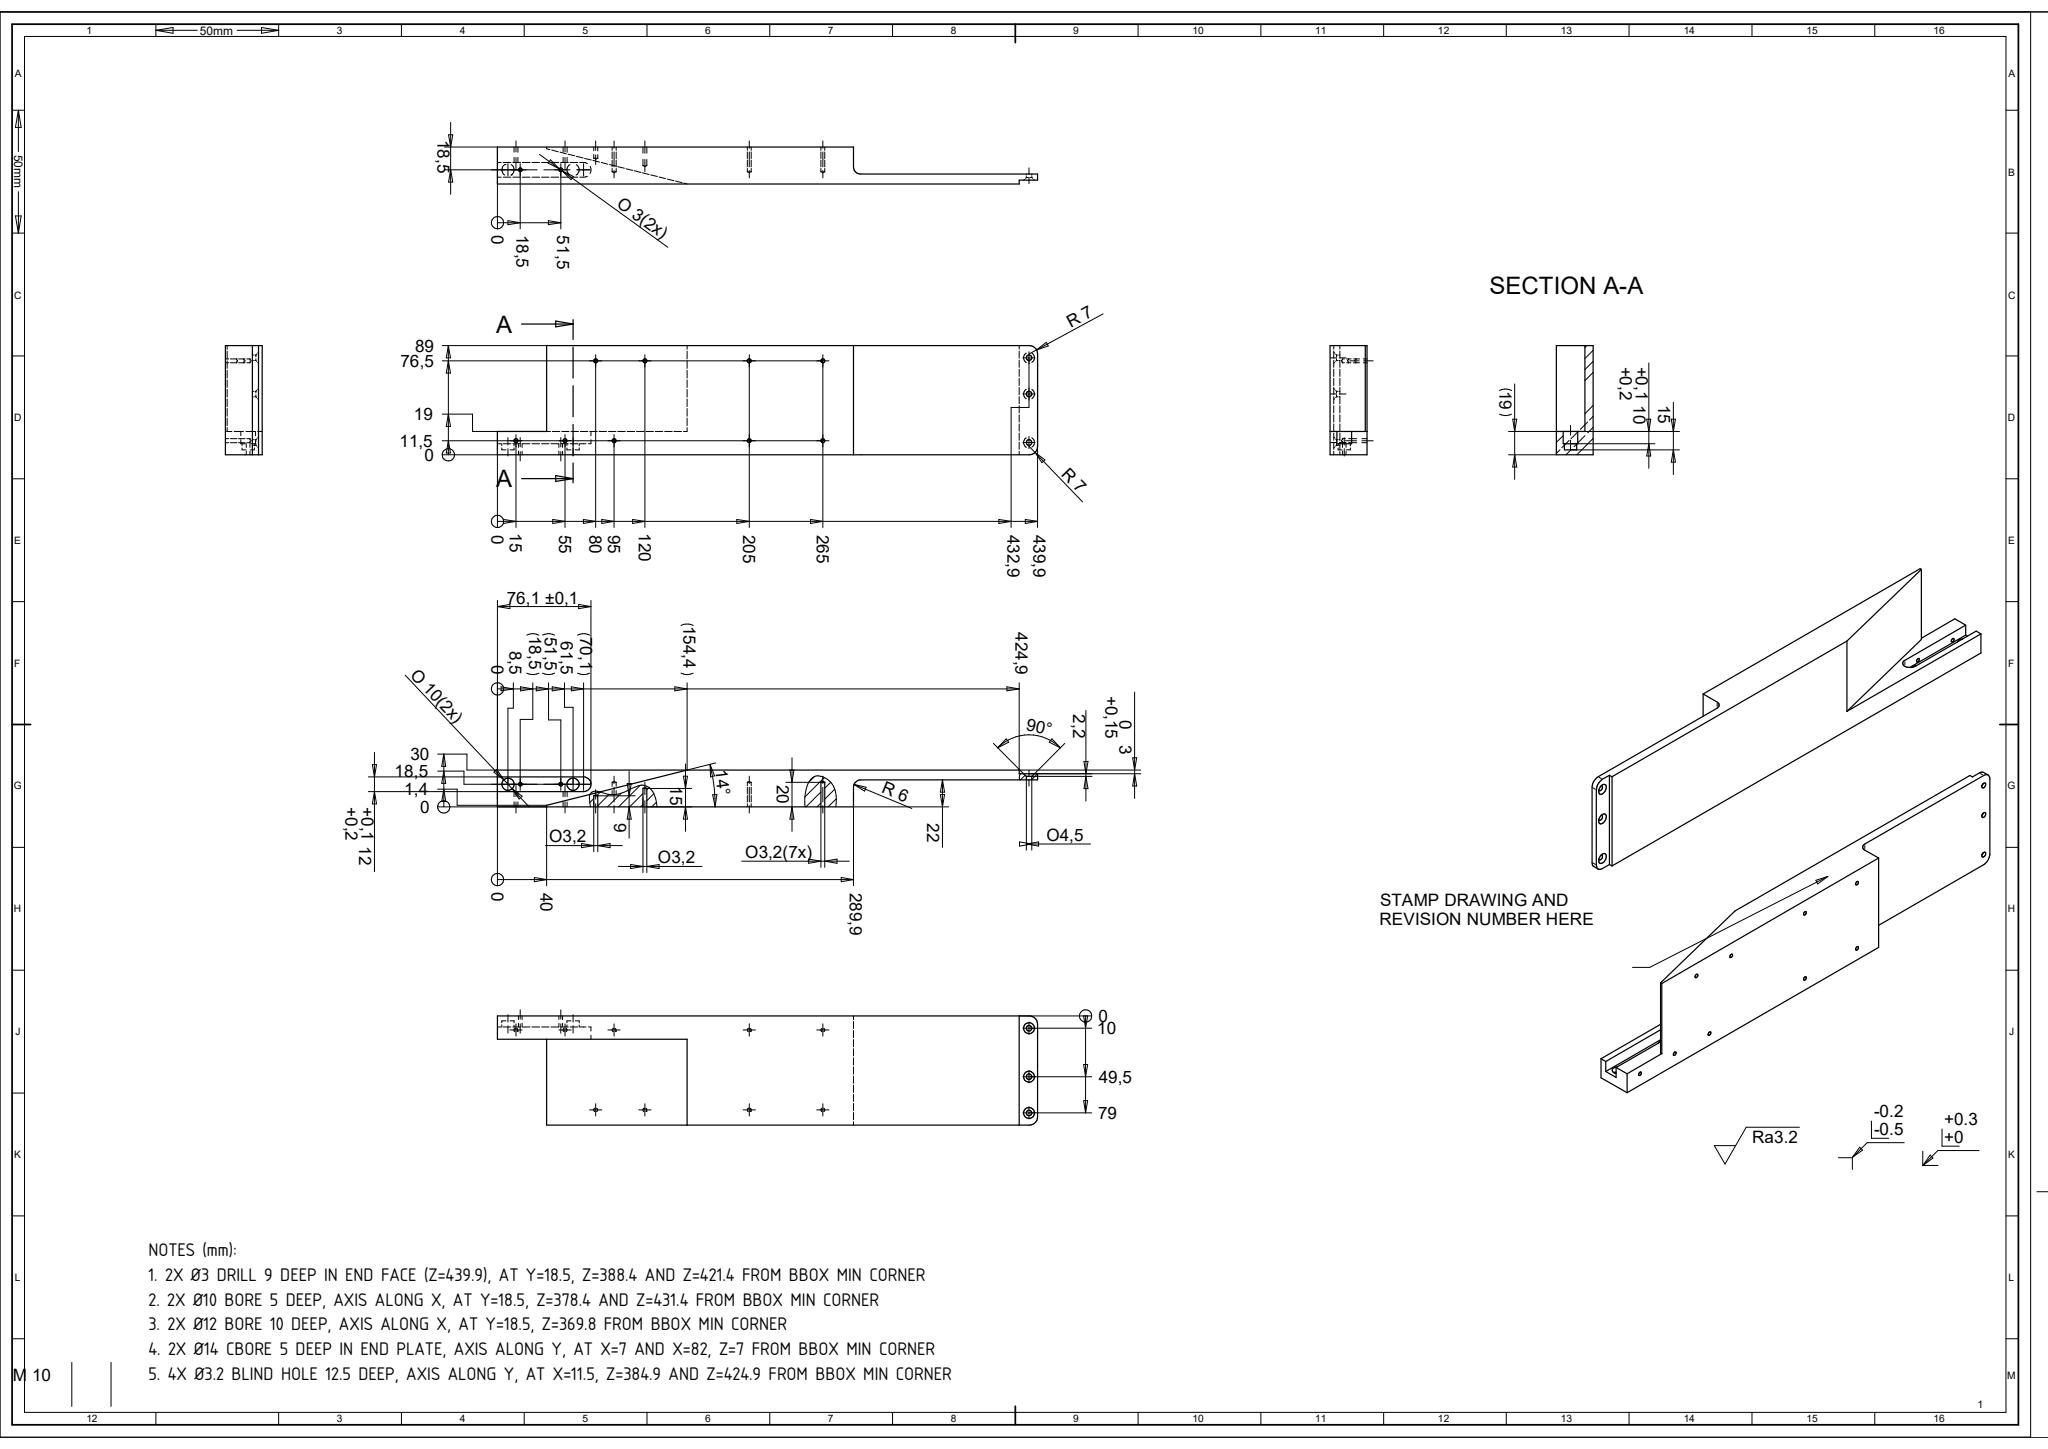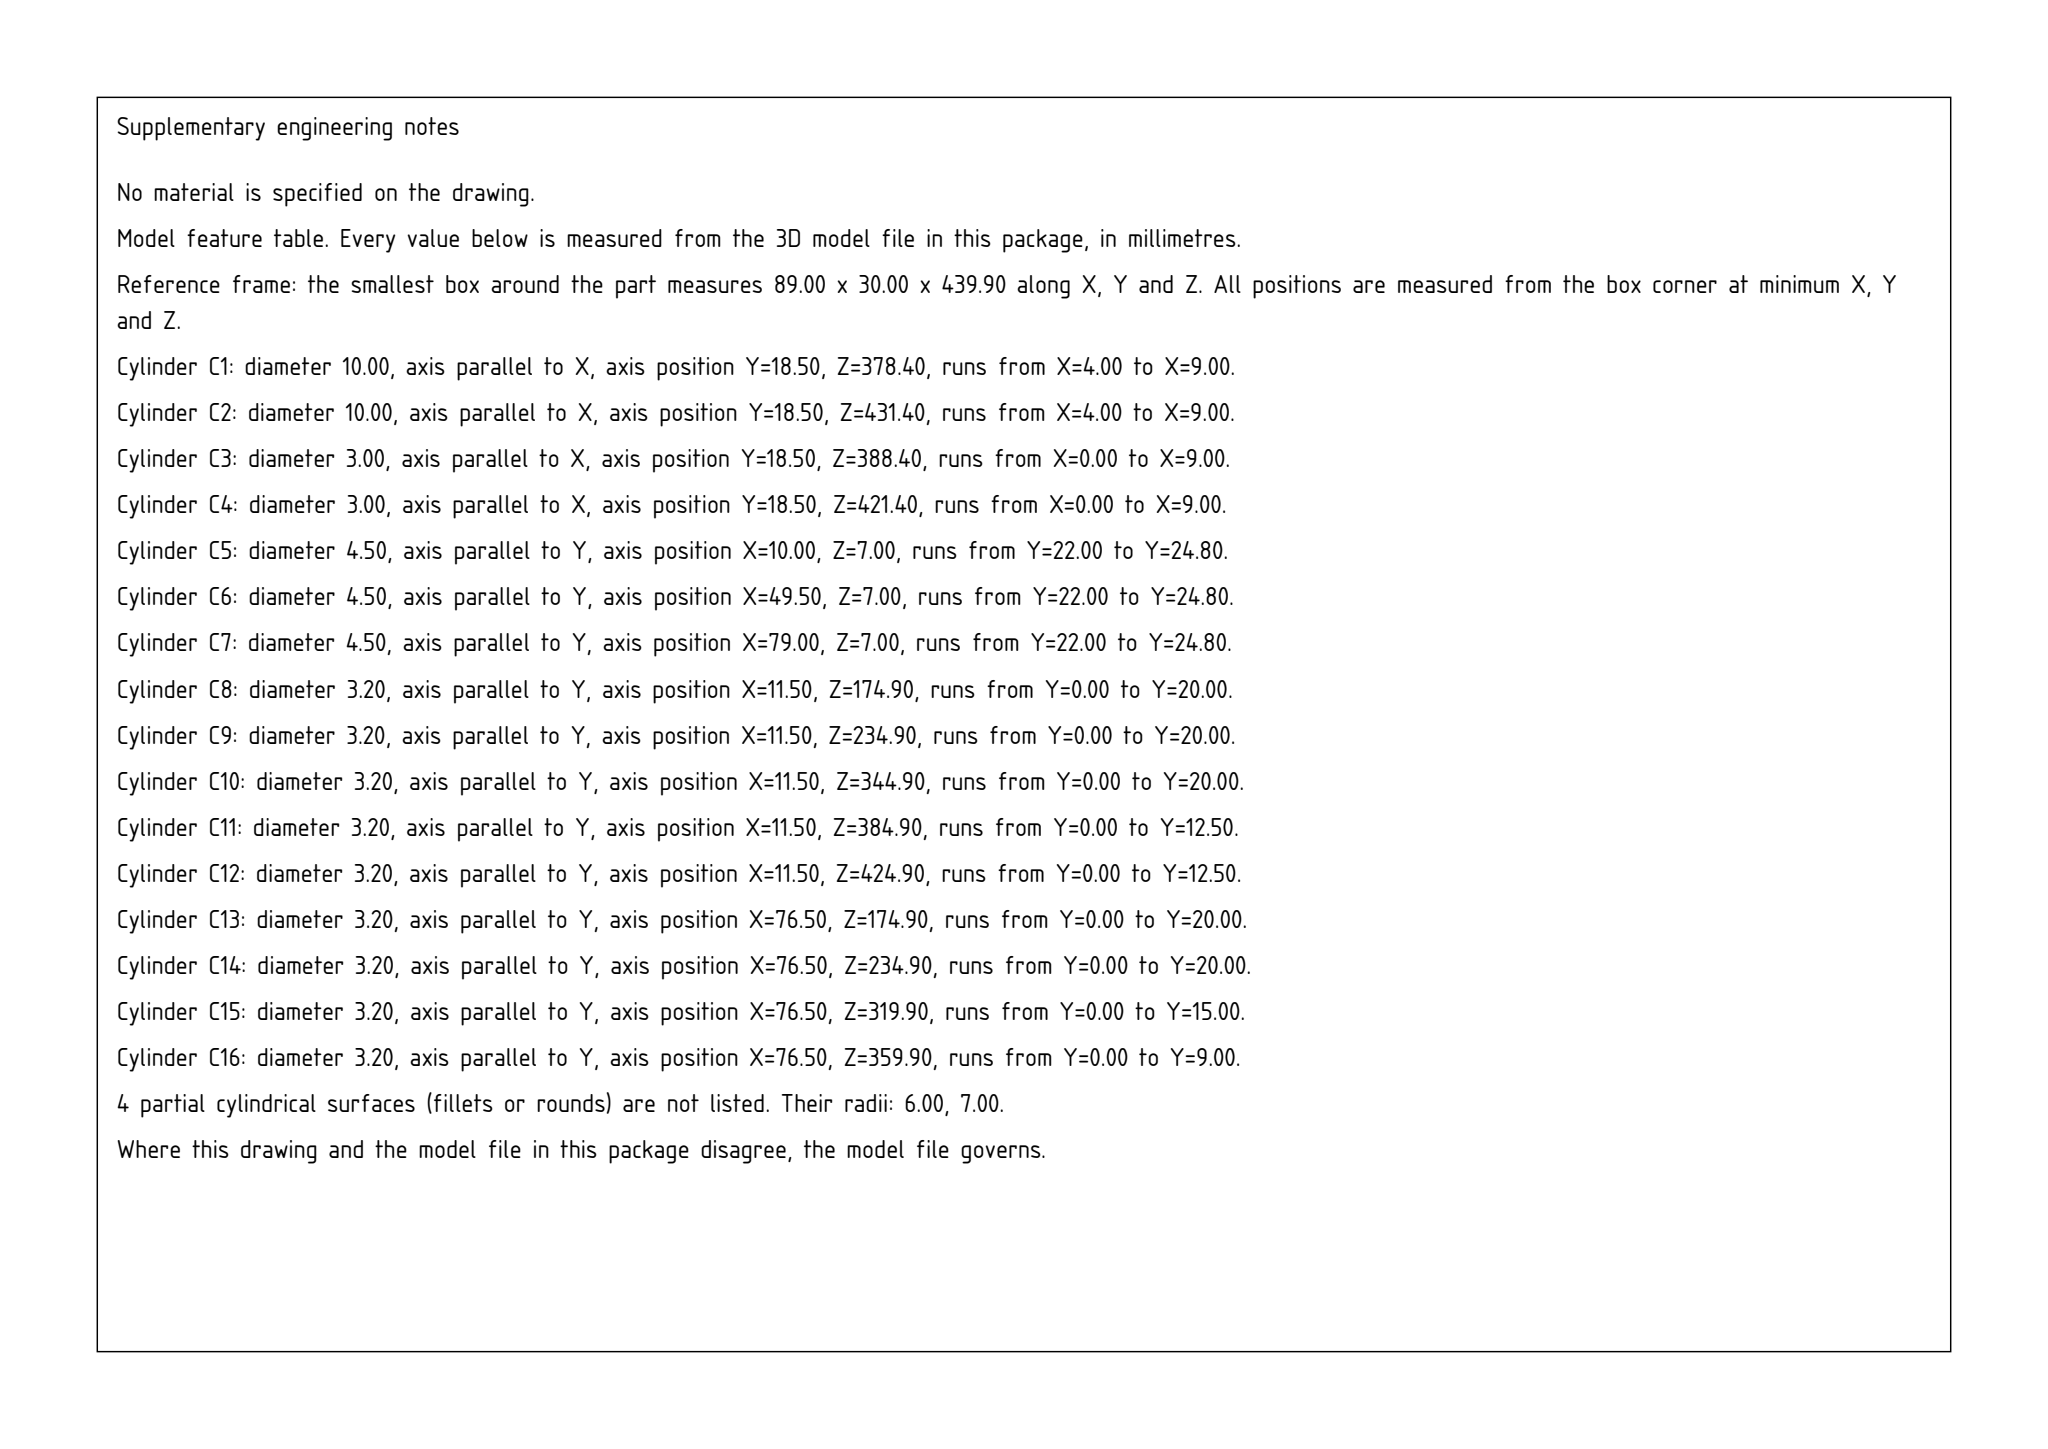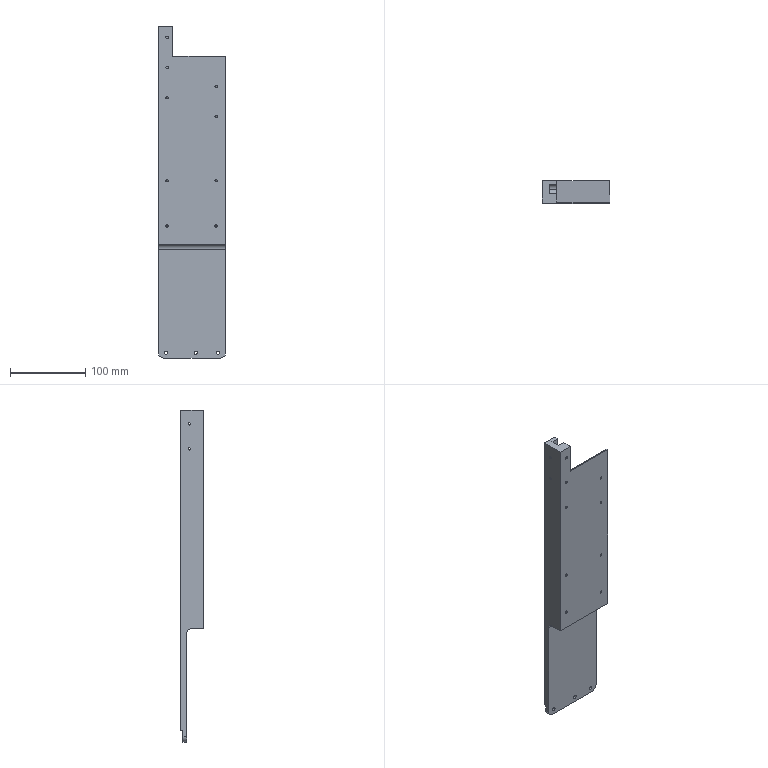Part | SolidWorks | mm | 1 solid | 75 faces | box 89 x 30 x 439.9 mm | volume 667415 mm3 | cylinder 37 | cone 20 | plane 18 | commonest cylinder face diameters 3.2 x18 4.5 x6 3 x4 10 x4 12 x3 14 x2
Drawing notes:
2X Ø3 DRILL 9 DEEP IN END FACE (Z=439.9), AT Y=18.5, Z=388.4 AND Z=421.4 FROM BBOX MIN CORNER | from the solid: cylinders [3.0,'x',[null,18.5,388.4],9.0] and [3.0,'x',[null,18.5,421.4],9.0]
2X Ø10 BORE 5 DEEP, AXIS ALONG X, AT Y=18.5, Z=378.4 AND Z=431.4 FROM BBOX MIN CORNER | from the solid: cylinders [10.0,'x',[null,18.5,378.4],5.0] and [10.0,'x',[null,18.5,431.4],5.0]
2X Ø12 BORE 10 DEEP, AXIS ALONG X, AT Y=18.5, Z=369.8 FROM BBOX MIN CORNER | from the solid: cylinder [12.0,'x',[null,18.5,369.8],10.0, count 2]
2X Ø14 CBORE 5 DEEP IN END PLATE, AXIS ALONG Y, AT X=7 AND X=82, Z=7 FROM BBOX MIN CORNER | from the solid: cylinders [14.0,'y',[7.0,null,7.0],5.0] and [14.0,'y',[82.0,null,7.0],5.0]
4X Ø3.2 BLIND HOLE 12.5 DEEP, AXIS ALONG Y, AT X=11.5, Z=384.9 AND Z=424.9 FROM BBOX MIN CORNER | from the solid: cylinders [3.2,'y',[11.5,null,384.9],12.5, count 2] and [3.2,'y',[11.5,null,424.9],12.5, count 2]